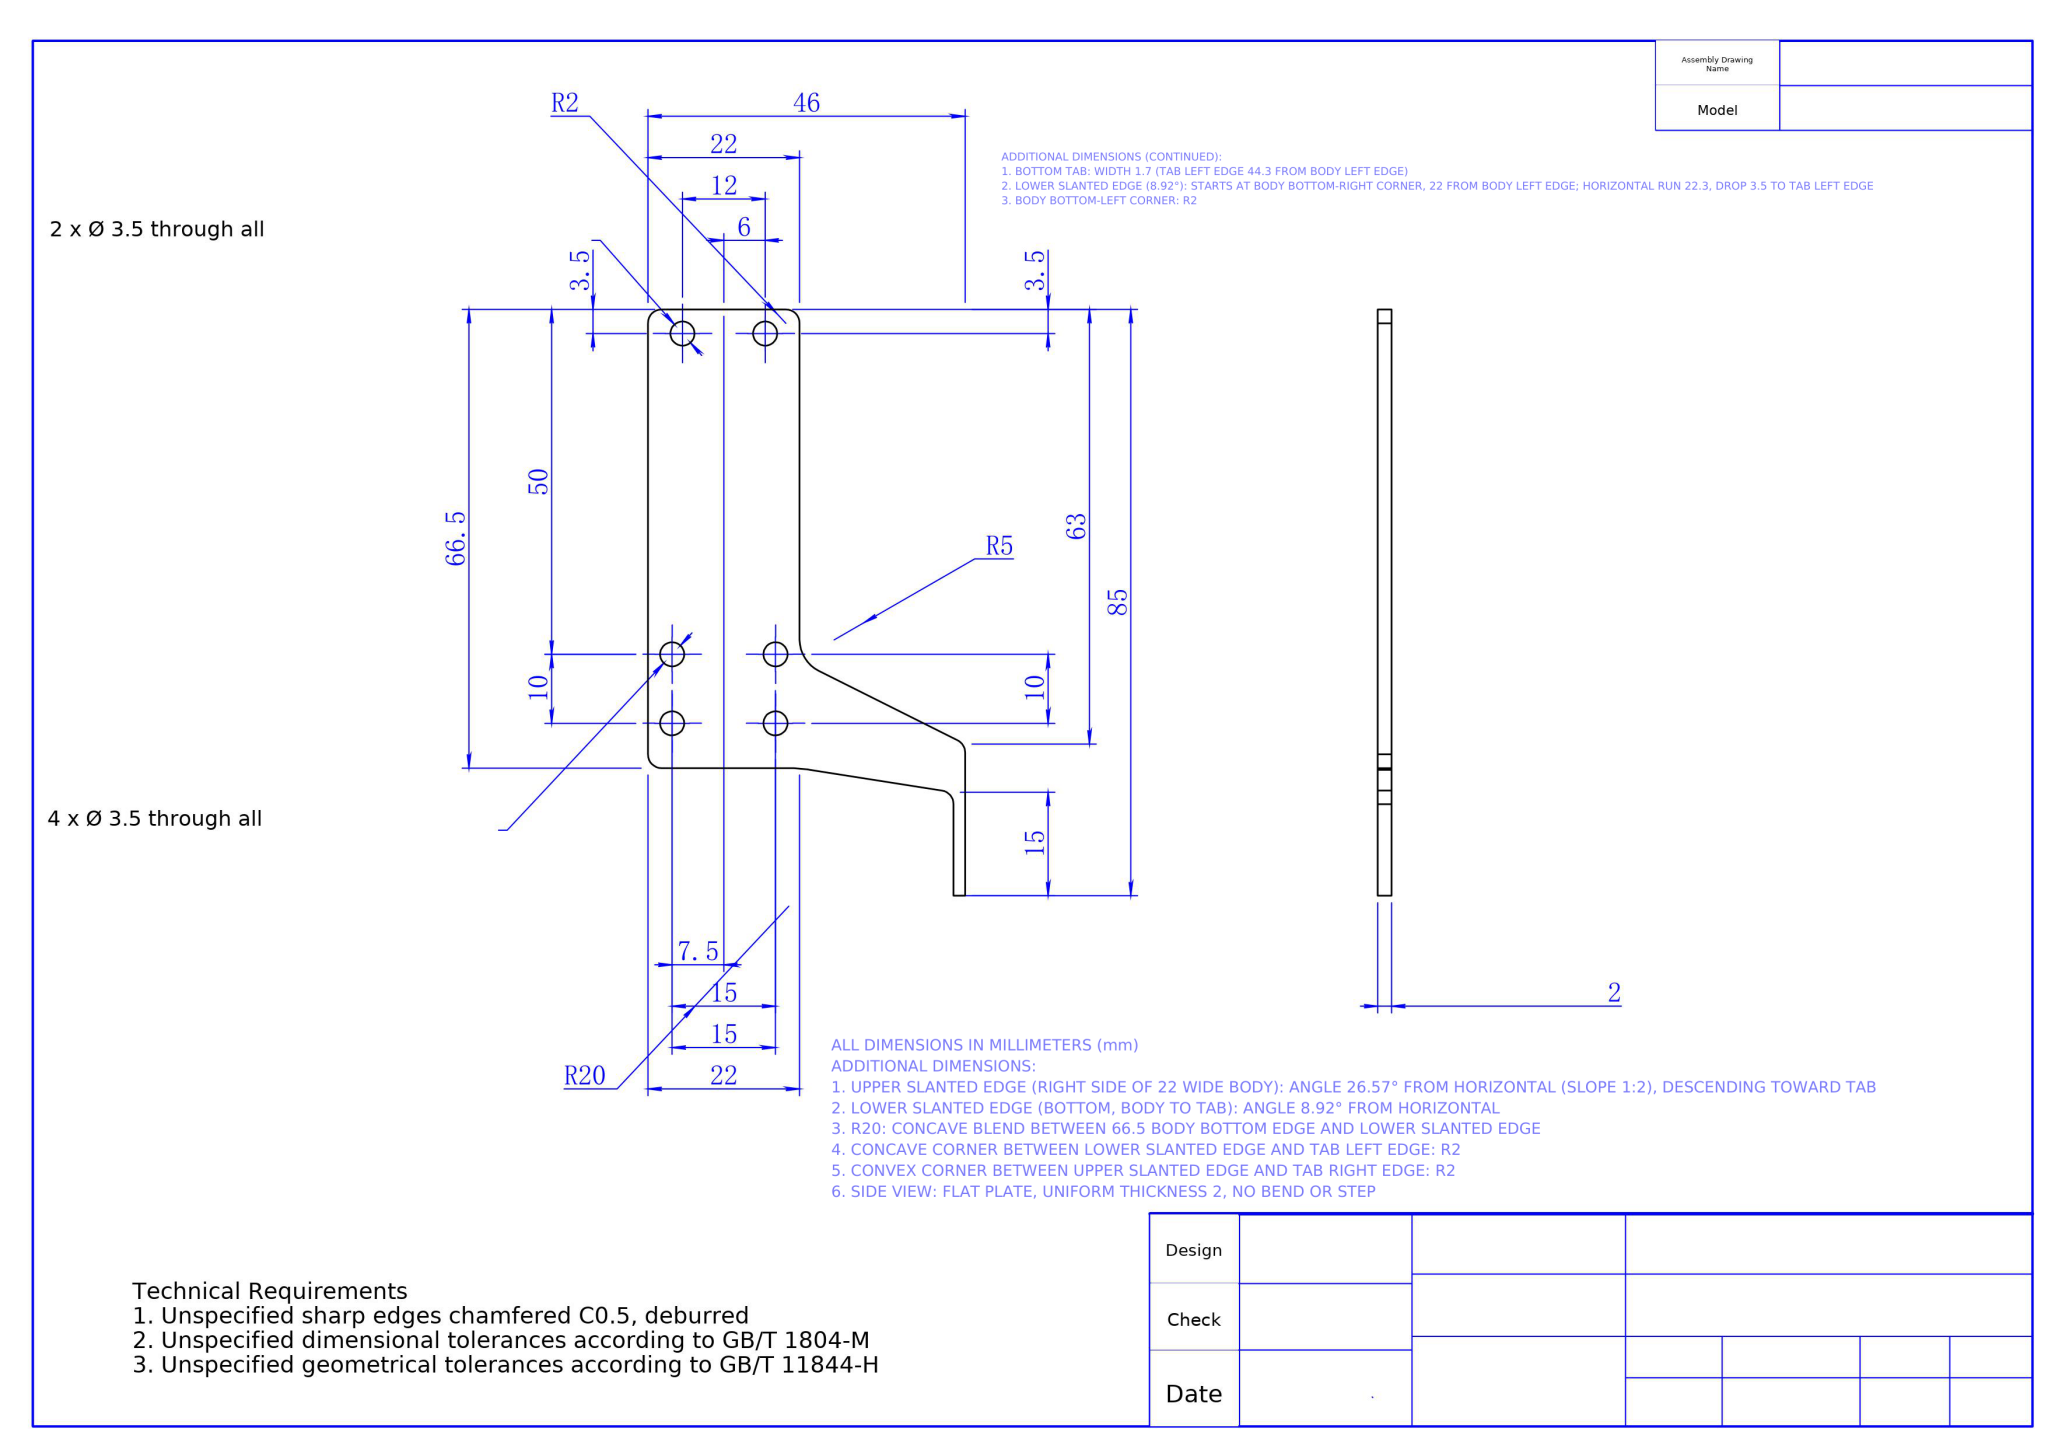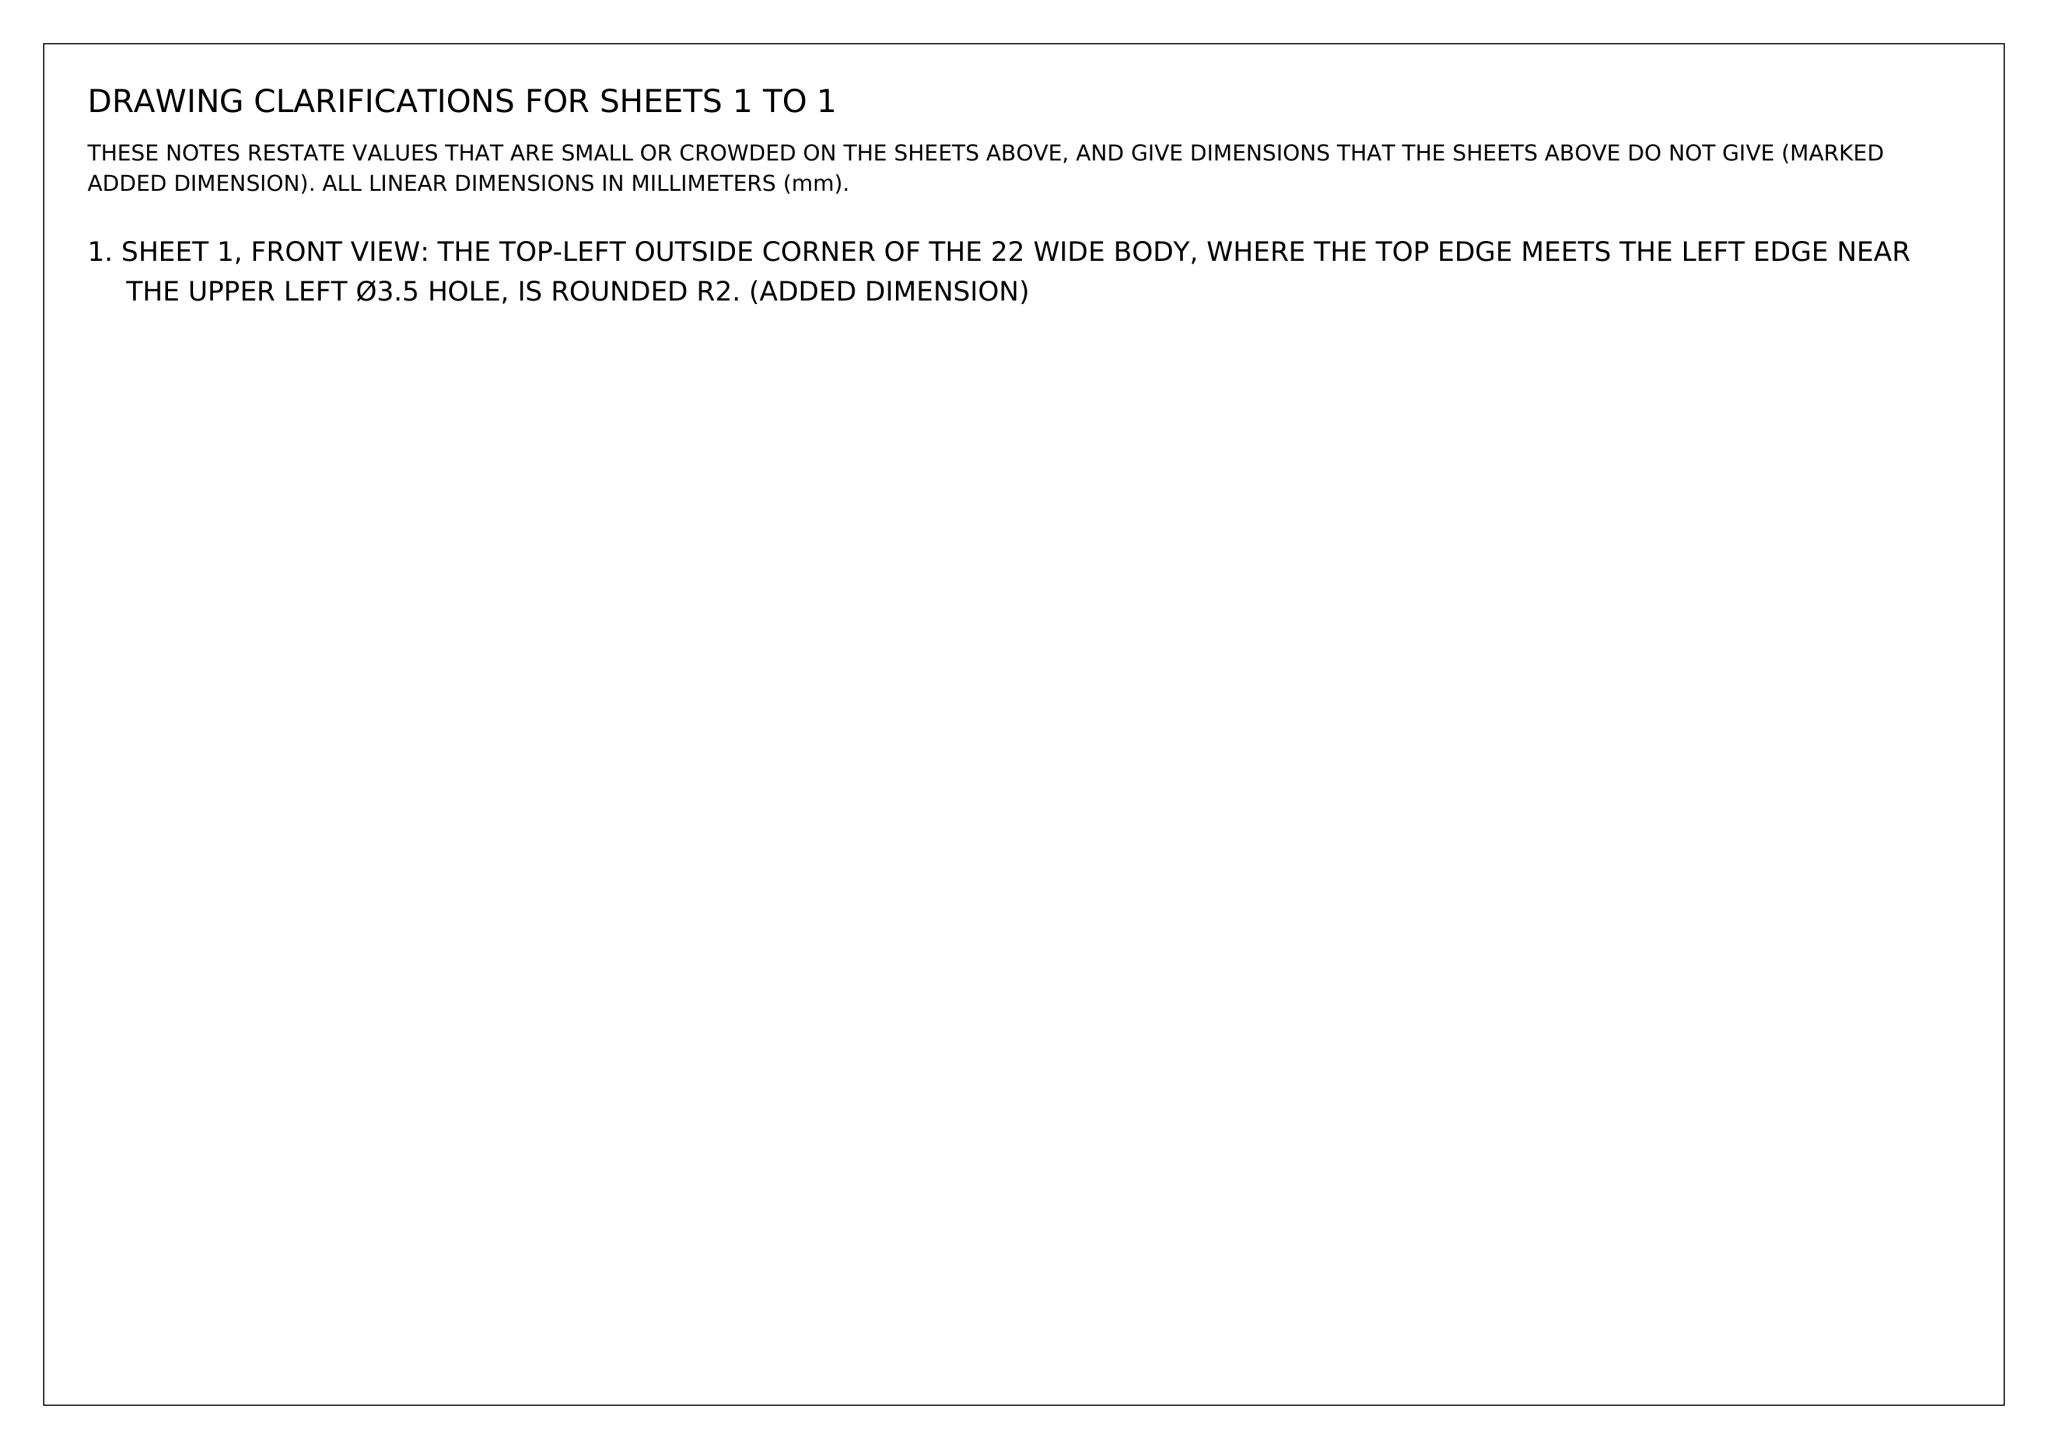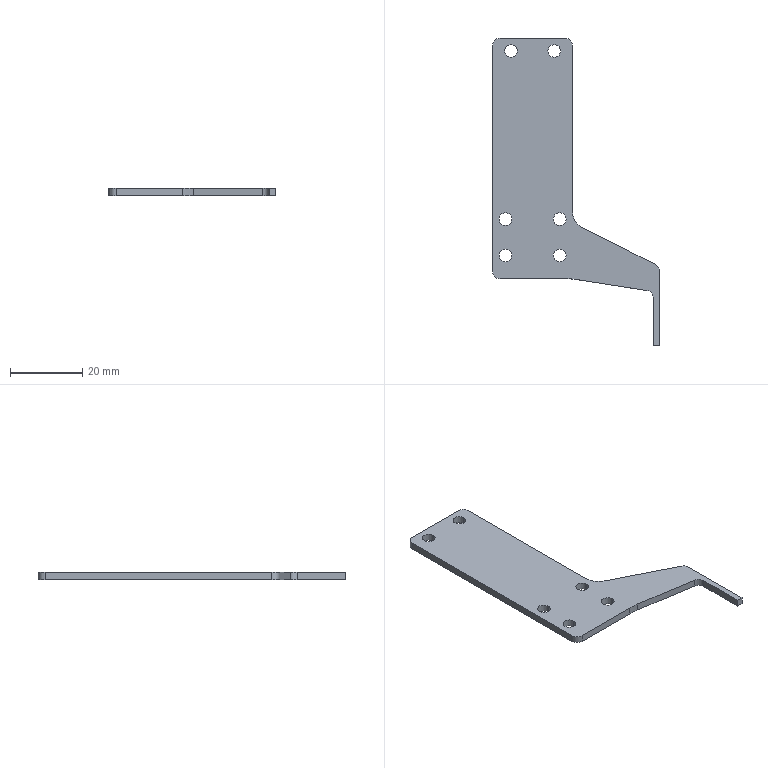Part | NX | mm | 1 solid | 30 faces | box 46 x 85 x 2 mm | volume 3406 mm3 | cylinder 19 | plane 11 | commonest cylinder face diameters 3.5 x12 4 x5 10 x1 40 x1